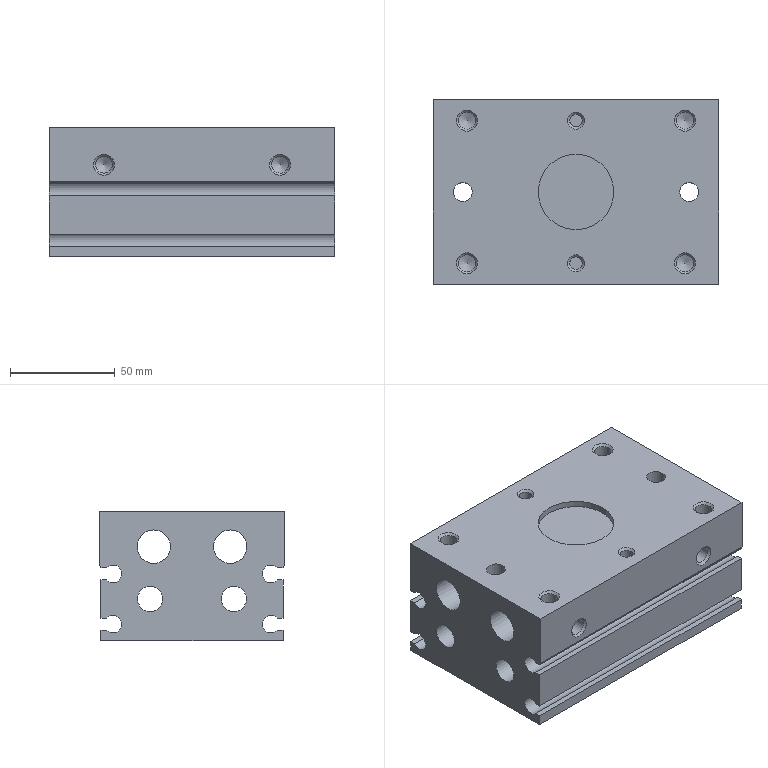Component | NX | CLAMP_CYL | 1 solid | 64 faces | volume 597868 mm3 | plane 25 | cylinder 21 | cone 18 | commonest cylinder face diameters 8 x8 8.4 x4 16 x2 12 x2 9 x2 6 x2 36 x1